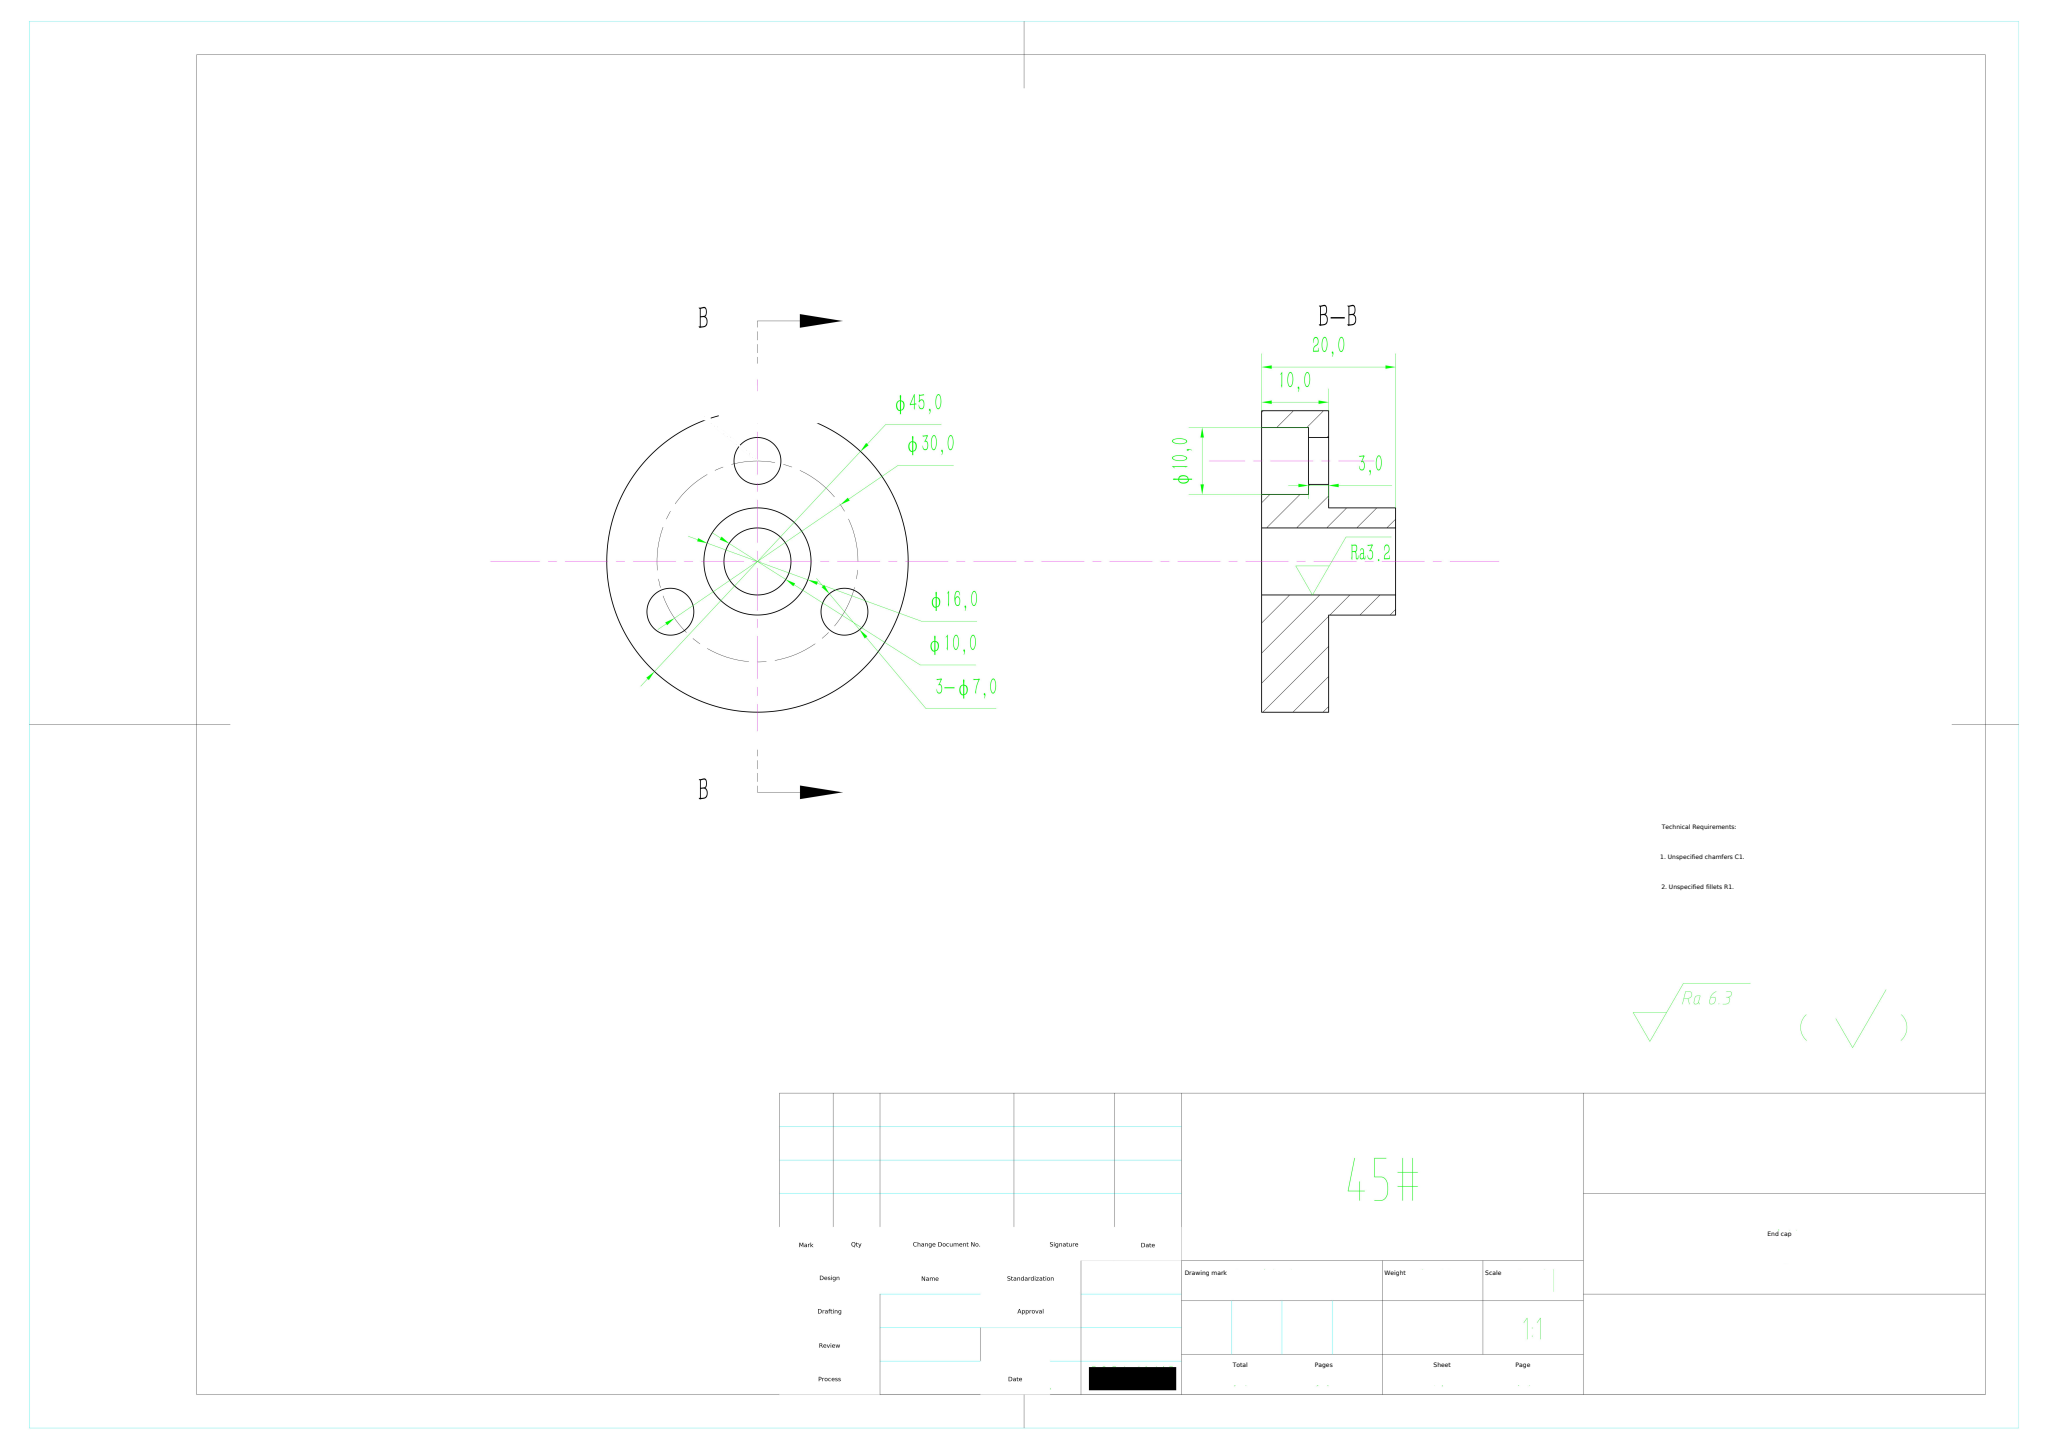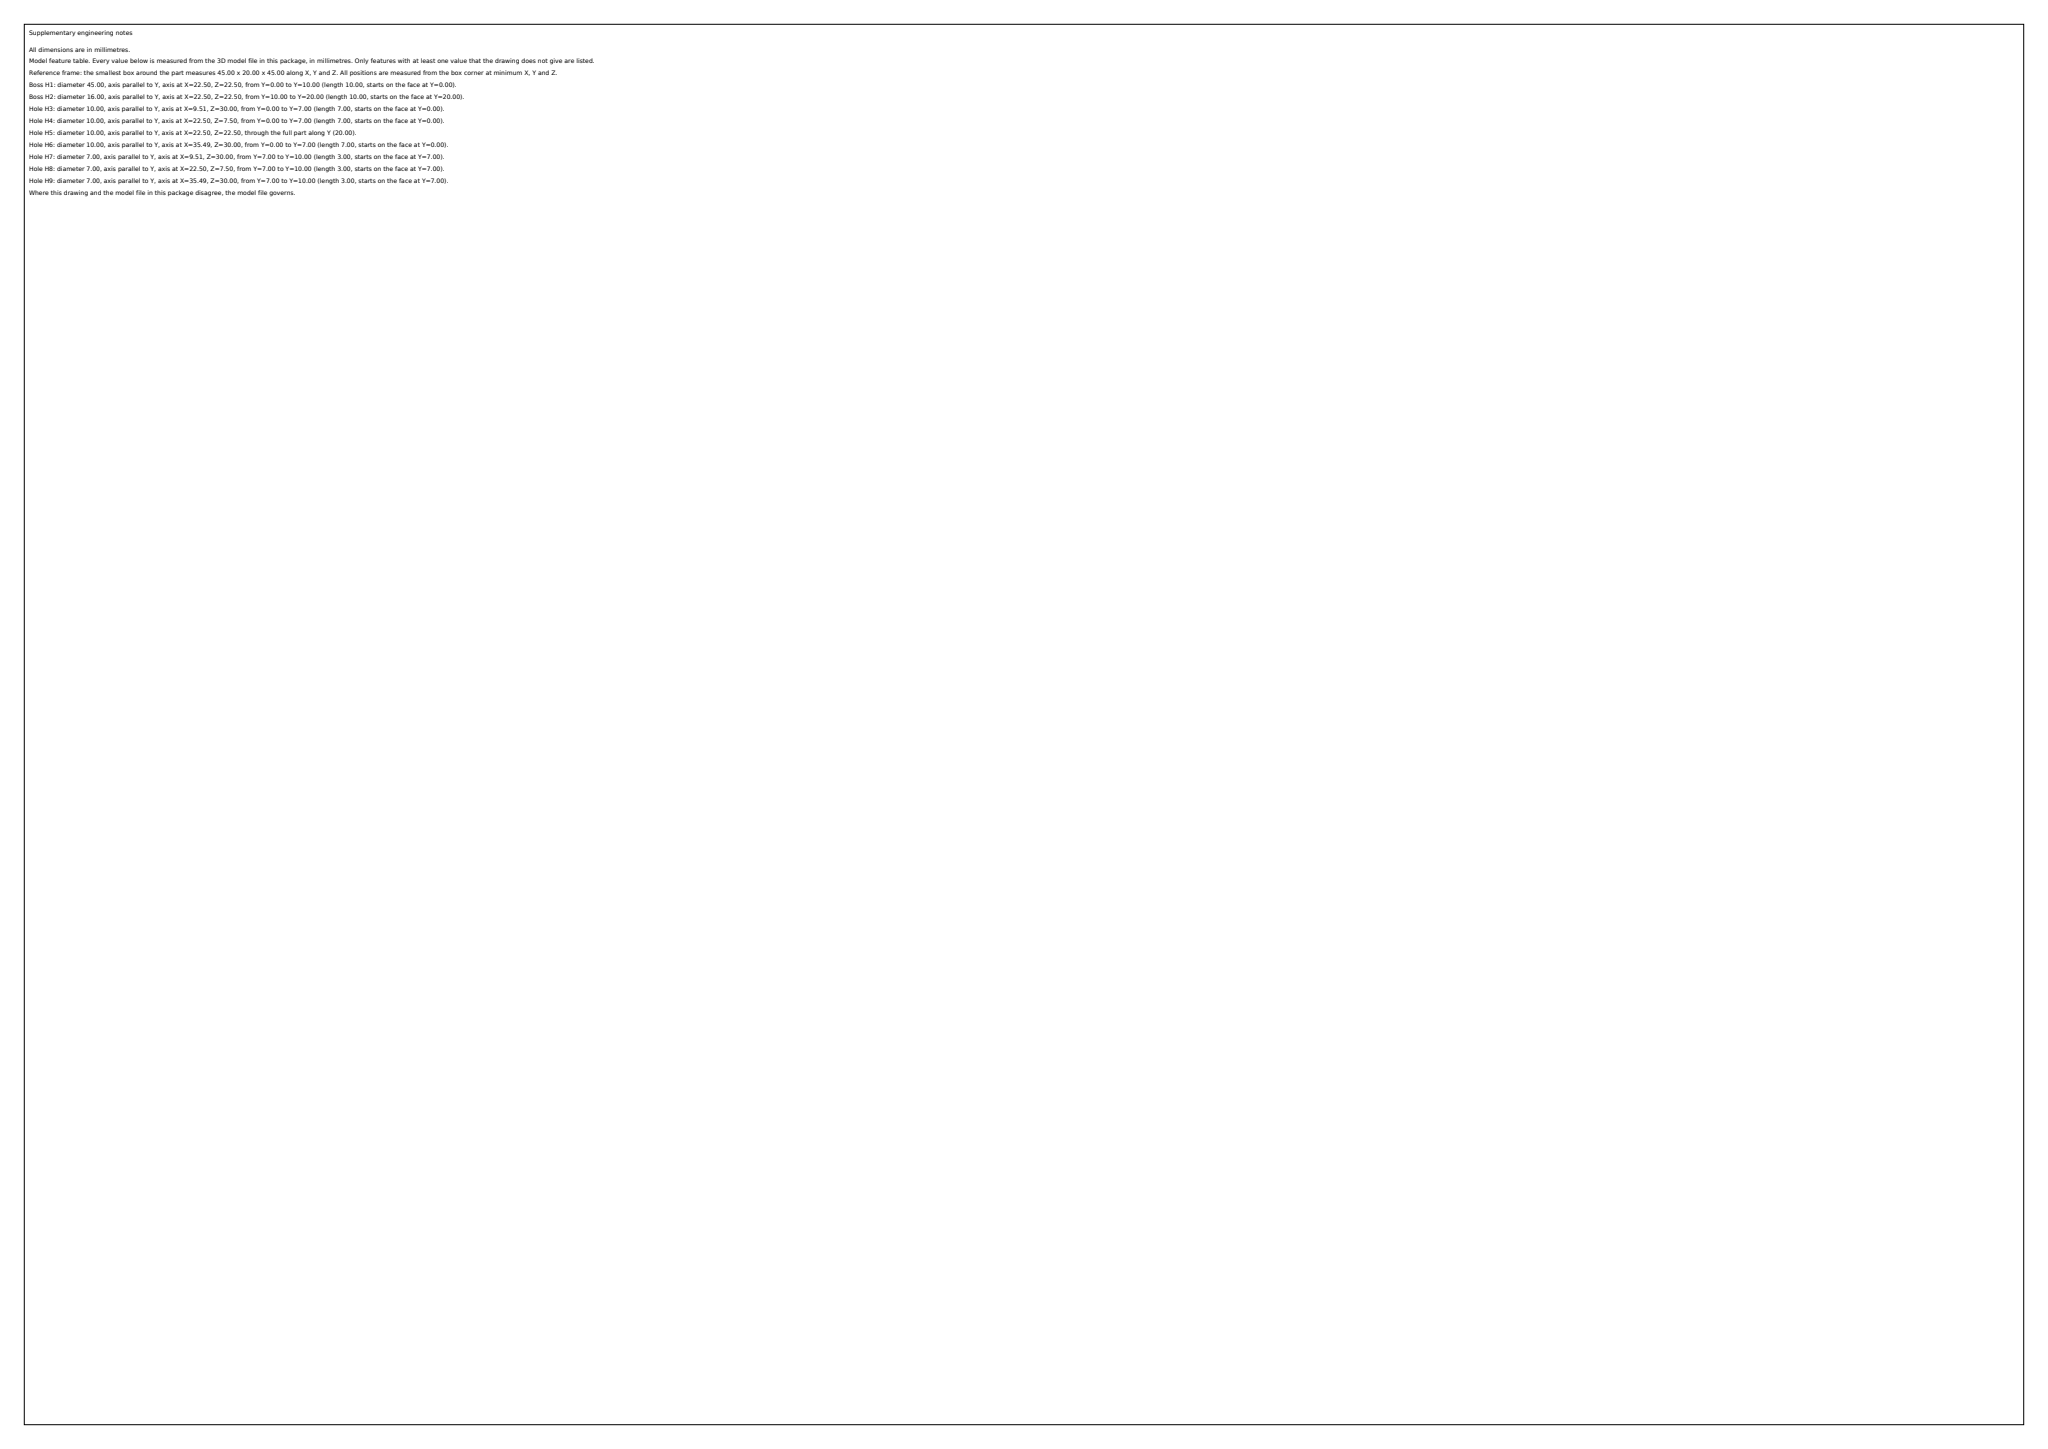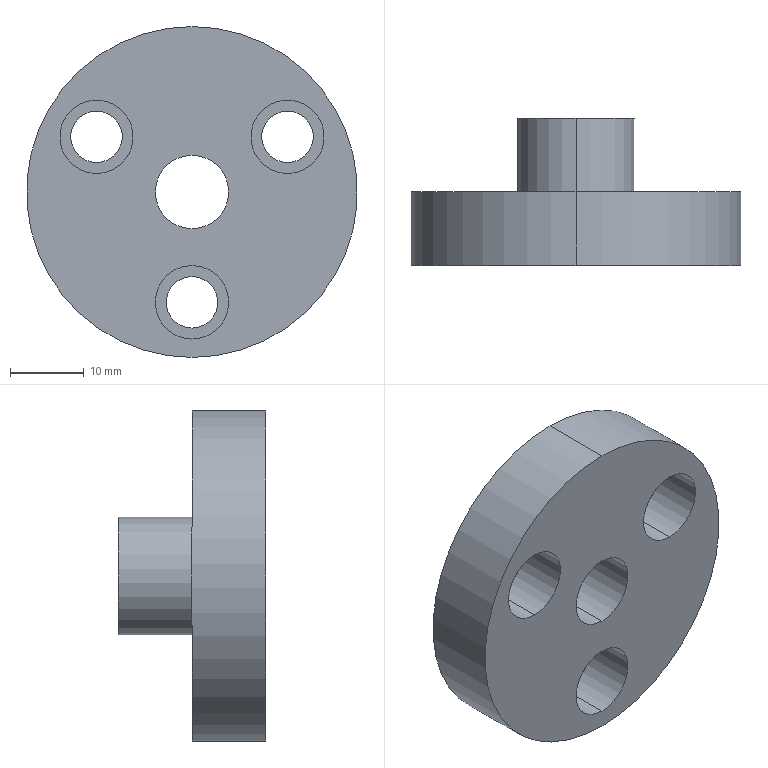Part | SolidWorks | mm | material 45# | 1 solid | 24 faces | box 45 x 20 x 45 mm | volume 14348 mm3 | cylinder 18 | plane 6 | commonest cylinder face diameters 10 x8 7 x6 16 x2 45 x2
build123d program:
from build123d import *

# Parameters (mm, degrees)
SKETCH1_R           = 22.5
BOSS_EXTRUDE1_DEPTH = 10
SKETCH2_R           = 8
BOSS_EXTRUDE2_DEPTH = 10
SKETCH3_R           = 3.5
CUT_EXTRUDE1_DEPTH  = 34.354
SKETCH4_R           = 5
CUT_EXTRUDE2_DEPTH  = 38.583
SKETCH5_R           = 5
CUT_EXTRUDE3_DEPTH  = 7


with BuildPart() as part:
    # Sketch1 → Boss-Extrude1 (new body)
    with BuildSketch(Plane(origin=(0, 0, 0), x_dir=(1, 0, 0), z_dir=(0, 1, 0))):
        with Locations(Location((0, 0, 0), (0, 0, 270))):
            Circle(SKETCH1_R)
    extrude(amount=BOSS_EXTRUDE1_DEPTH)

    # Sketch2 → Boss-Extrude2 (add)
    with BuildSketch(Plane(origin=(0, 10, 0), x_dir=(1, 0, 0), z_dir=(0, 1, 0))):
        with Locations(Location((0, 0, 0), (0, 0, 270))):
            Circle(SKETCH2_R)
    extrude(amount=BOSS_EXTRUDE2_DEPTH)

    # Sketch3 → Cut-Extrude1 (cut, through all)
    with BuildSketch(Plane(origin=(0, 10, 0), x_dir=(1, 0, 0), z_dir=(0, 1, 0))):
        with Locations(Location((0, 15, 0), (0, 0, 270))):
            Circle(SKETCH3_R)
        with Locations(Location((12.99, -7.5, 0), (0, 0, 270))):
            Circle(SKETCH3_R)
        with Locations(Location((-12.99, -7.5, 0), (0, 0, 270))):
            Circle(SKETCH3_R)
    extrude(amount=-CUT_EXTRUDE1_DEPTH, mode=Mode.SUBTRACT)

    # Sketch4 → Cut-Extrude2 (cut, through all)
    with BuildSketch(Plane(origin=(0, 20, 0), x_dir=(1, 0, 0), z_dir=(0, 1, 0))):
        with Locations(Location((0, 0, 0), (0, 0, 270))):
            Circle(SKETCH4_R)
    extrude(amount=-CUT_EXTRUDE2_DEPTH, mode=Mode.SUBTRACT)

    # Sketch5 → Cut-Extrude3 (cut)
    with BuildSketch(Plane.XZ):
        with Locations(Location((12.99, 7.5, 0), (0, 0, 270))):
            Circle(SKETCH5_R)
        with Locations(Location((0, -15, 0), (0, 0, 270))):
            Circle(SKETCH5_R)
        with Locations(Location((-12.99, 7.5, 0), (0, 0, 270))):
            Circle(SKETCH5_R)
    extrude(amount=-CUT_EXTRUDE3_DEPTH, mode=Mode.SUBTRACT)


solid = part.part
STEP:
#1=CARTESIAN_POINT('',(-12.99,7.,12.5));
#2=VERTEX_POINT('',#1);
#3=CARTESIAN_POINT('',(-12.99,7.,2.5));
#4=VERTEX_POINT('',#3);
#5=CARTESIAN_POINT('',(-12.99,7.,7.5));
#6=DIRECTION('',(0.,-1.,0.));
#7=DIRECTION('',(0.,0.,-1.));
#8=AXIS2_PLACEMENT_3D('',#5,#6,#7);
#9=CIRCLE('',#8,5.);
#10=EDGE_CURVE('',#2,#4,#9,.T.);
#11=ORIENTED_EDGE('',*,*,#10,.F.);
#12=CARTESIAN_POINT('',(-12.99,0.,12.5));
#13=VERTEX_POINT('',#12);
#14=CARTESIAN_POINT('',(-12.99,7.,12.5));
#15=DIRECTION('',(0.,-1.,0.));
#16=VECTOR('',#15,1000.);
#17=LINE('',#14,#16);
#18=EDGE_CURVE('',#2,#13,#17,.T.);
#19=ORIENTED_EDGE('',*,*,#18,.T.);
#20=CARTESIAN_POINT('',(-12.99,0.,2.5));
#21=VERTEX_POINT('',#20);
#22=CARTESIAN_POINT('',(-12.99,0.,7.5));
#23=DIRECTION('',(0.,-1.,0.));
#24=DIRECTION('',(0.,0.,-1.));
#25=AXIS2_PLACEMENT_3D('',#22,#23,#24);
#26=CIRCLE('',#25,5.);
#27=EDGE_CURVE('',#13,#21,#26,.T.);
#28=ORIENTED_EDGE('',*,*,#27,.T.);
#29=CARTESIAN_POINT('',(-12.99,7.,2.5));
#30=DIRECTION('',(0.,-1.,0.));
#31=VECTOR('',#30,1000.);
#32=LINE('',#29,#31);
#33=EDGE_CURVE('',#4,#21,#32,.T.);
#34=ORIENTED_EDGE('',*,*,#33,.F.);
#35=EDGE_LOOP('',(#11,#19,#28,#34));
#36=FACE_OUTER_BOUND('',#35,.T.);
#37=CARTESIAN_POINT('',(-12.99,7.,7.5));
#38=DIRECTION('',(0.,-1.,0.));
#39=DIRECTION('',(0.,0.,-1.));
#40=AXIS2_PLACEMENT_3D('',#37,#38,#39);
#41=CYLINDRICAL_SURFACE('',#40,5.);
#42=ADVANCED_FACE('',(#36),#41,.F.);
#43=CARTESIAN_POINT('',(12.99,7.,12.5));
#44=VERTEX_POINT('',#43);
#45=CARTESIAN_POINT('',(12.99,7.,2.5));
#46=VERTEX_POINT('',#45);
#47=CARTESIAN_POINT('',(12.99,7.,7.5));
#48=DIRECTION('',(0.,-1.,0.));
#49=DIRECTION('',(0.,0.,-1.));
#50=AXIS2_PLACEMENT_3D('',#47,#48,#49);
#51=CIRCLE('',#50,5.);
#52=EDGE_CURVE('',#44,#46,#51,.T.);
#53=ORIENTED_EDGE('',*,*,#52,.F.);
#54=CARTESIAN_POINT('',(12.99,0.,12.5));
#55=VERTEX_POINT('',#54);
#56=CARTESIAN_POINT('',(12.99,7.,12.5));
#57=DIRECTION('',(0.,-1.,0.));
#58=VECTOR('',#57,1000.);
#59=LINE('',#56,#58);
#60=EDGE_CURVE('',#44,#55,#59,.T.);
#61=ORIENTED_EDGE('',*,*,#60,.T.);
#62=CARTESIAN_POINT('',(12.99,0.,2.5));
#63=VERTEX_POINT('',#62);
#64=CARTESIAN_POINT('',(12.99,0.,7.5));
#65=DIRECTION('',(0.,-1.,0.));
#66=DIRECTION('',(0.,0.,-1.));
#67=AXIS2_PLACEMENT_3D('',#64,#65,#66);
#68=CIRCLE('',#67,5.);
#69=EDGE_CURVE('',#55,#63,#68,.T.);
#70=ORIENTED_EDGE('',*,*,#69,.T.);
#71=CARTESIAN_POINT('',(12.99,7.,2.5));
#72=DIRECTION('',(0.,-1.,0.));
#73=VECTOR('',#72,1000.);
#74=LINE('',#71,#73);
#75=EDGE_CURVE('',#46,#63,#74,.T.);
#76=ORIENTED_EDGE('',*,*,#75,.F.);
#77=EDGE_LOOP('',(#53,#61,#70,#76));
#78=FACE_OUTER_BOUND('',#77,.T.);
#79=CARTESIAN_POINT('',(12.99,7.,7.5));
#80=DIRECTION('',(0.,-1.,0.));
#81=DIRECTION('',(0.,0.,-1.));
#82=AXIS2_PLACEMENT_3D('',#79,#80,#81);
#83=CYLINDRICAL_SURFACE('',#82,5.);
#84=ADVANCED_FACE('',(#78),#83,.F.);
#85=CARTESIAN_POINT('',(-0.,7.,-10.));
#86=VERTEX_POINT('',#85);
#87=CARTESIAN_POINT('',(-0.,7.,-20.));
#88=VERTEX_POINT('',#87);
#89=CARTESIAN_POINT('',(-0.,7.,-15.));
#90=DIRECTION('',(0.,-1.,0.));
#91=DIRECTION('',(0.,0.,-1.));
#92=AXIS2_PLACEMENT_3D('',#89,#90,#91);
#93=CIRCLE('',#92,5.);
#94=EDGE_CURVE('',#86,#88,#93,.T.);
#95=ORIENTED_EDGE('',*,*,#94,.F.);
#96=CARTESIAN_POINT('',(-0.,0.,-10.));
#97=VERTEX_POINT('',#96);
#98=CARTESIAN_POINT('',(-0.,7.,-10.));
#99=DIRECTION('',(0.,-1.,0.));
#100=VECTOR('',#99,1000.);
#101=LINE('',#98,#100);
#102=EDGE_CURVE('',#86,#97,#101,.T.);
#103=ORIENTED_EDGE('',*,*,#102,.T.);
#104=CARTESIAN_POINT('',(-0.,0.,-20.));
#105=VERTEX_POINT('',#104);
#106=CARTESIAN_POINT('',(-0.,0.,-15.));
#107=DIRECTION('',(0.,-1.,0.));
#108=DIRECTION('',(0.,0.,-1.));
#109=AXIS2_PLACEMENT_3D('',#106,#107,#108);
#110=CIRCLE('',#109,5.);
#111=EDGE_CURVE('',#97,#105,#110,.T.);
#112=ORIENTED_EDGE('',*,*,#111,.T.);
#113=CARTESIAN_POINT('',(-0.,7.,-20.));
#114=DIRECTION('',(0.,-1.,0.));
#115=VECTOR('',#114,1000.);
#116=LINE('',#113,#115);
#117=EDGE_CURVE('',#88,#105,#116,.T.);
#118=ORIENTED_EDGE('',*,*,#117,.F.);
#119=EDGE_LOOP('',(#95,#103,#112,#118));
#120=FACE_OUTER_BOUND('',#119,.T.);
#121=CARTESIAN_POINT('',(-0.,7.,-15.));
#122=DIRECTION('',(0.,-1.,0.));
#123=DIRECTION('',(0.,0.,-1.));
#124=AXIS2_PLACEMENT_3D('',#121,#122,#123);
#125=CYLINDRICAL_SURFACE('',#124,5.);
#126=ADVANCED_FACE('',(#120),#125,.F.);
#127=CARTESIAN_POINT('',(0.,0.,-5.));
#128=VERTEX_POINT('',#127);
#129=CARTESIAN_POINT('',(0.,0.,5.));
#130=VERTEX_POINT('',#129);
#131=CARTESIAN_POINT('',(0.,0.,0.));
#132=DIRECTION('',(0.,1.,0.));
#133=DIRECTION('',(0.,0.,1.));
#134=AXIS2_PLACEMENT_3D('',#131,#132,#133);
#135=CIRCLE('',#134,5.);
#136=EDGE_CURVE('',#128,#130,#135,.T.);
#137=ORIENTED_EDGE('',*,*,#136,.F.);
#138=CARTESIAN_POINT('',(0.,20.,-5.));
#139=VERTEX_POINT('',#138);
#140=CARTESIAN_POINT('',(0.,0.,-5.));
#141=DIRECTION('',(0.,1.,0.));
#142=VECTOR('',#141,1000.);
#143=LINE('',#140,#142);
#144=EDGE_CURVE('',#128,#139,#143,.T.);
#145=ORIENTED_EDGE('',*,*,#144,.T.);
#146=CARTESIAN_POINT('',(0.,20.,5.));
#147=VERTEX_POINT('',#146);
#148=CARTESIAN_POINT('',(0.,20.,0.));
#149=DIRECTION('',(0.,1.,0.));
#150=DIRECTION('',(0.,0.,1.));
#151=AXIS2_PLACEMENT_3D('',#148,#149,#150);
#152=CIRCLE('',#151,5.);
#153=EDGE_CURVE('',#139,#147,#152,.T.);
#154=ORIENTED_EDGE('',*,*,#153,.T.);
#155=CARTESIAN_POINT('',(0.,0.,5.));
#156=DIRECTION('',(0.,1.,0.));
#157=VECTOR('',#156,1000.);
#158=LINE('',#155,#157);
#159=EDGE_CURVE('',#130,#147,#158,.T.);
#160=ORIENTED_EDGE('',*,*,#159,.F.);
#161=EDGE_LOOP('',(#137,#145,#154,#160));
#162=FACE_OUTER_BOUND('',#161,.T.);
#163=CARTESIAN_POINT('',(0.,0.,0.));
#164=DIRECTION('',(0.,1.,0.));
#165=DIRECTION('',(0.,0.,1.));
#166=AXIS2_PLACEMENT_3D('',#163,#164,#165);
#167=CYLINDRICAL_SURFACE('',#166,5.);
#168=ADVANCED_FACE('',(#162),#167,.F.);
#169=CARTESIAN_POINT('',(0.,20.,8.));
#170=VERTEX_POINT('',#169);
#171=CARTESIAN_POINT('',(0.,20.,-8.));
#172=VERTEX_POINT('',#171);
#173=CARTESIAN_POINT('',(0.,20.,0.));
#174=DIRECTION('',(0.,1.,0.));
#175=DIRECTION('',(0.,0.,1.));
#176=AXIS2_PLACEMENT_3D('',#173,#174,#175);
#177=CIRCLE('',#176,8.);
#178=EDGE_CURVE('',#170,#172,#177,.T.);
#179=ORIENTED_EDGE('',*,*,#178,.F.);
#180=CARTESIAN_POINT('',(0.,10.,8.));
#181=VERTEX_POINT('',#180);
#182=CARTESIAN_POINT('',(0.,20.,8.));
#183=DIRECTION('',(0.,-1.,0.));
#184=VECTOR('',#183,1000.);
#185=LINE('',#182,#184);
#186=EDGE_CURVE('',#170,#181,#185,.T.);
#187=ORIENTED_EDGE('',*,*,#186,.T.);
#188=CARTESIAN_POINT('',(0.,10.,-8.));
#189=VERTEX_POINT('',#188);
#190=CARTESIAN_POINT('',(0.,10.,0.));
#191=DIRECTION('',(0.,1.,0.));
#192=DIRECTION('',(0.,0.,1.));
#193=AXIS2_PLACEMENT_3D('',#190,#191,#192);
#194=CIRCLE('',#193,8.);
#195=EDGE_CURVE('',#181,#189,#194,.T.);
#196=ORIENTED_EDGE('',*,*,#195,.T.);
#197=CARTESIAN_POINT('',(0.,20.,-8.));
#198=DIRECTION('',(0.,-1.,0.));
#199=VECTOR('',#198,1000.);
#200=LINE('',#197,#199);
#201=EDGE_CURVE('',#172,#189,#200,.T.);
#202=ORIENTED_EDGE('',*,*,#201,.F.);
#203=EDGE_LOOP('',(#179,#187,#196,#202));
#204=FACE_OUTER_BOUND('',#203,.T.);
#205=CARTESIAN_POINT('',(0.,20.,0.));
#206=DIRECTION('',(0.,-1.,0.));
#207=DIRECTION('',(0.,0.,-1.));
#208=AXIS2_PLACEMENT_3D('',#205,#206,#207);
#209=CYLINDRICAL_SURFACE('',#208,8.);
#210=ADVANCED_FACE('',(#204),#209,.T.);
#211=CARTESIAN_POINT('',(0.,10.,22.5));
#212=VERTEX_POINT('',#211);
#213=CARTESIAN_POINT('',(0.,10.,-22.5));
#214=VERTEX_POINT('',#213);
#215=CARTESIAN_POINT('',(0.,10.,0.));
#216=DIRECTION('',(0.,1.,0.));
#217=DIRECTION('',(0.,0.,1.));
#218=AXIS2_PLACEMENT_3D('',#215,#216,#217);
#219=CIRCLE('',#218,22.5);
#220=EDGE_CURVE('',#212,#214,#219,.T.);
#221=ORIENTED_EDGE('',*,*,#220,.F.);
#222=CARTESIAN_POINT('',(0.,0.,22.5));
#223=VERTEX_POINT('',#222);
#224=CARTESIAN_POINT('',(0.,10.,22.5));
#225=DIRECTION('',(0.,-1.,0.));
#226=VECTOR('',#225,1000.);
#227=LINE('',#224,#226);
#228=EDGE_CURVE('',#212,#223,#227,.T.);
#229=ORIENTED_EDGE('',*,*,#228,.T.);
#230=CARTESIAN_POINT('',(0.,0.,-22.5));
#231=VERTEX_POINT('',#230);
#232=CARTESIAN_POINT('',(0.,0.,0.));
#233=DIRECTION('',(0.,1.,0.));
#234=DIRECTION('',(0.,0.,1.));
#235=AXIS2_PLACEMENT_3D('',#232,#233,#234);
#236=CIRCLE('',#235,22.5);
#237=EDGE_CURVE('',#223,#231,#236,.T.);
#238=ORIENTED_EDGE('',*,*,#237,.T.);
#239=CARTESIAN_POINT('',(0.,10.,-22.5));
#240=DIRECTION('',(0.,-1.,0.));
#241=VECTOR('',#240,1000.);
#242=LINE('',#239,#241);
#243=EDGE_CURVE('',#214,#231,#242,.T.);
#244=ORIENTED_EDGE('',*,*,#243,.F.);
#245=EDGE_LOOP('',(#221,#229,#238,#244));
#246=FACE_OUTER_BOUND('',#245,.T.);
#247=CARTESIAN_POINT('',(0.,10.,0.));
#248=DIRECTION('',(0.,-1.,0.));
#249=DIRECTION('',(0.,0.,-1.));
#250=AXIS2_PLACEMENT_3D('',#247,#248,#249);
#251=CYLINDRICAL_SURFACE('',#250,22.5);
#252=ADVANCED_FACE('',(#246),#251,.T.);
#253=CARTESIAN_POINT('',(0.,7.,-18.5));
#254=VERTEX_POINT('',#253);
#255=CARTESIAN_POINT('',(0.,7.,-11.5));
#256=VERTEX_POINT('',#255);
#257=CARTESIAN_POINT('',(0.,7.,-15.));
#258=DIRECTION('',(0.,1.,0.));
#259=DIRECTION('',(0.,0.,-1.));
#260=AXIS2_PLACEMENT_3D('',#257,#258,#259);
#261=CIRCLE('',#260,3.5);
#262=EDGE_CURVE('',#254,#256,#261,.T.);
#263=ORIENTED_EDGE('',*,*,#262,.F.);
#264=CARTESIAN_POINT('',(0.,10.,-18.5));
#265=VERTEX_POINT('',#264);
#266=CARTESIAN_POINT('',(0.,0.,-18.5));
#267=DIRECTION('',(0.,1.,0.));
#268=VECTOR('',#267,1000.);
#269=LINE('',#266,#268);
#270=EDGE_CURVE('',#254,#265,#269,.T.);
#271=ORIENTED_EDGE('',*,*,#270,.T.);
#272=CARTESIAN_POINT('',(0.,10.,-11.5));
#273=VERTEX_POINT('',#272);
#274=CARTESIAN_POINT('',(0.,10.,-15.));
#275=DIRECTION('',(0.,1.,0.));
#276=DIRECTION('',(0.,0.,1.));
#277=AXIS2_PLACEMENT_3D('',#274,#275,#276);
#278=CIRCLE('',#277,3.5);
#279=EDGE_CURVE('',#265,#273,#278,.T.);
#280=ORIENTED_EDGE('',*,*,#279,.T.);
#281=CARTESIAN_POINT('',(0.,0.,-11.5));
#282=DIRECTION('',(0.,1.,0.));
#283=VECTOR('',#282,1000.);
#284=LINE('',#281,#283);
#285=EDGE_CURVE('',#256,#273,#284,.T.);
#286=ORIENTED_EDGE('',*,*,#285,.F.);
#287=EDGE_LOOP('',(#263,#271,#280,#286));
#288=FACE_OUTER_BOUND('',#287,.T.);
#289=CARTESIAN_POINT('',(0.,0.,-15.));
#290=DIRECTION('',(0.,1.,0.));
#291=DIRECTION('',(0.,0.,1.));
#292=AXIS2_PLACEMENT_3D('',#289,#290,#291);
#293=CYLINDRICAL_SURFACE('',#292,3.5);
#294=ADVANCED_FACE('',(#288),#293,.F.);
#295=CARTESIAN_POINT('',(12.99,7.,4.));
#296=VERTEX_POINT('',#295);
#297=CARTESIAN_POINT('',(12.99,7.,11.));
#298=VERTEX_POINT('',#297);
#299=CARTESIAN_POINT('',(12.99,7.,7.5));
#300=DIRECTION('',(0.,1.,0.));
#301=DIRECTION('',(0.,0.,-1.));
#302=AXIS2_PLACEMENT_3D('',#299,#300,#301);
#303=CIRCLE('',#302,3.5);
#304=EDGE_CURVE('',#296,#298,#303,.T.);
#305=ORIENTED_EDGE('',*,*,#304,.F.);
#306=CARTESIAN_POINT('',(12.99,10.,4.));
#307=VERTEX_POINT('',#306);
#308=CARTESIAN_POINT('',(12.99,0.,4.));
#309=DIRECTION('',(0.,1.,0.));
#310=VECTOR('',#309,1000.);
#311=LINE('',#308,#310);
#312=EDGE_CURVE('',#296,#307,#311,.T.);
#313=ORIENTED_EDGE('',*,*,#312,.T.);
#314=CARTESIAN_POINT('',(12.99,10.,11.));
#315=VERTEX_POINT('',#314);
#316=CARTESIAN_POINT('',(12.99,10.,7.5));
#317=DIRECTION('',(0.,1.,0.));
#318=DIRECTION('',(0.,0.,1.));
#319=AXIS2_PLACEMENT_3D('',#316,#317,#318);
#320=CIRCLE('',#319,3.5);
#321=EDGE_CURVE('',#307,#315,#320,.T.);
#322=ORIENTED_EDGE('',*,*,#321,.T.);
#323=CARTESIAN_POINT('',(12.99,0.,11.));
#324=DIRECTION('',(0.,1.,0.));
#325=VECTOR('',#324,1000.);
#326=LINE('',#323,#325);
#327=EDGE_CURVE('',#298,#315,#326,.T.);
#328=ORIENTED_EDGE('',*,*,#327,.F.);
#329=EDGE_LOOP('',(#305,#313,#322,#328));
#330=FACE_OUTER_BOUND('',#329,.T.);
#331=CARTESIAN_POINT('',(12.99,0.,7.5));
#332=DIRECTION('',(0.,1.,0.));
#333=DIRECTION('',(0.,0.,1.));
#334=AXIS2_PLACEMENT_3D('',#331,#332,#333);
#335=CYLINDRICAL_SURFACE('',#334,3.5);
#336=ADVANCED_FACE('',(#330),#335,.F.);
#337=CARTESIAN_POINT('',(-12.99,7.,4.));
#338=VERTEX_POINT('',#337);
#339=CARTESIAN_POINT('',(-12.99,7.,11.));
#340=VERTEX_POINT('',#339);
#341=CARTESIAN_POINT('',(-12.99,7.,7.5));
#342=DIRECTION('',(0.,1.,0.));
#343=DIRECTION('',(0.,0.,-1.));
#344=AXIS2_PLACEMENT_3D('',#341,#342,#343);
#345=CIRCLE('',#344,3.5);
#346=EDGE_CURVE('',#338,#340,#345,.T.);
#347=ORIENTED_EDGE('',*,*,#346,.F.);
#348=CARTESIAN_POINT('',(-12.99,10.,4.));
#349=VERTEX_POINT('',#348);
#350=CARTESIAN_POINT('',(-12.99,0.,4.));
#351=DIRECTION('',(0.,1.,0.));
#352=VECTOR('',#351,1000.);
#353=LINE('',#350,#352);
#354=EDGE_CURVE('',#338,#349,#353,.T.);
#355=ORIENTED_EDGE('',*,*,#354,.T.);
#356=CARTESIAN_POINT('',(-12.99,10.,11.));
#357=VERTEX_POINT('',#356);
#358=CARTESIAN_POINT('',(-12.99,10.,7.5));
#359=DIRECTION('',(0.,1.,0.));
#360=DIRECTION('',(0.,0.,1.));
#361=AXIS2_PLACEMENT_3D('',#358,#359,#360);
#362=CIRCLE('',#361,3.5);
#363=EDGE_CURVE('',#349,#357,#362,.T.);
#364=ORIENTED_EDGE('',*,*,#363,.T.);
#365=CARTESIAN_POINT('',(-12.99,0.,11.));
#366=DIRECTION('',(0.,1.,0.));
#367=VECTOR('',#366,1000.);
#368=LINE('',#365,#367);
#369=EDGE_CURVE('',#340,#357,#368,.T.);
#370=ORIENTED_EDGE('',*,*,#369,.F.);
#371=EDGE_LOOP('',(#347,#355,#364,#370));
#372=FACE_OUTER_BOUND('',#371,.T.);
#373=CARTESIAN_POINT('',(-12.99,0.,7.5));
#374=DIRECTION('',(0.,1.,0.));
#375=DIRECTION('',(0.,0.,1.));
#376=AXIS2_PLACEMENT_3D('',#373,#374,#375);
#377=CYLINDRICAL_SURFACE('',#376,3.5);
#378=ADVANCED_FACE('',(#372),#377,.F.);
#379=ORIENTED_EDGE('',*,*,#354,.F.);
#380=CARTESIAN_POINT('',(-12.99,7.,7.5));
#381=DIRECTION('',(0.,1.,0.));
#382=DIRECTION('',(0.,0.,-1.));
#383=AXIS2_PLACEMENT_3D('',#380,#381,#382);
#384=CIRCLE('',#383,3.5);
#385=EDGE_CURVE('',#340,#338,#384,.T.);
#386=ORIENTED_EDGE('',*,*,#385,.F.);
#387=ORIENTED_EDGE('',*,*,#369,.T.);
#388=CARTESIAN_POINT('',(-12.99,10.,7.5));
#389=DIRECTION('',(0.,1.,0.));
#390=DIRECTION('',(0.,0.,1.));
#391=AXIS2_PLACEMENT_3D('',#388,#389,#390);
#392=CIRCLE('',#391,3.5);
#393=EDGE_CURVE('',#357,#349,#392,.T.);
#394=ORIENTED_EDGE('',*,*,#393,.T.);
#395=EDGE_LOOP('',(#379,#386,#387,#394));
#396=FACE_OUTER_BOUND('',#395,.T.);
#397=CARTESIAN_POINT('',(-12.99,0.,7.5));
#398=DIRECTION('',(0.,1.,0.));
#399=DIRECTION('',(0.,0.,1.));
#400=AXIS2_PLACEMENT_3D('',#397,#398,#399);
#401=CYLINDRICAL_SURFACE('',#400,3.5);
#402=ADVANCED_FACE('',(#396),#401,.F.);
#403=ORIENTED_EDGE('',*,*,#312,.F.);
#404=CARTESIAN_POINT('',(12.99,7.,7.5));
#405=DIRECTION('',(0.,1.,0.));
#406=DIRECTION('',(0.,0.,-1.));
#407=AXIS2_PLACEMENT_3D('',#404,#405,#406);
#408=CIRCLE('',#407,3.5);
#409=EDGE_CURVE('',#298,#296,#408,.T.);
#410=ORIENTED_EDGE('',*,*,#409,.F.);
#411=ORIENTED_EDGE('',*,*,#327,.T.);
#412=CARTESIAN_POINT('',(12.99,10.,7.5));
#413=DIRECTION('',(0.,1.,0.));
#414=DIRECTION('',(0.,0.,1.));
#415=AXIS2_PLACEMENT_3D('',#412,#413,#414);
#416=CIRCLE('',#415,3.5);
#417=EDGE_CURVE('',#315,#307,#416,.T.);
#418=ORIENTED_EDGE('',*,*,#417,.T.);
#419=EDGE_LOOP('',(#403,#410,#411,#418));
#420=FACE_OUTER_BOUND('',#419,.T.);
#421=CARTESIAN_POINT('',(12.99,0.,7.5));
#422=DIRECTION('',(0.,1.,0.));
#423=DIRECTION('',(0.,0.,1.));
#424=AXIS2_PLACEMENT_3D('',#421,#422,#423);
#425=CYLINDRICAL_SURFACE('',#424,3.5);
#426=ADVANCED_FACE('',(#420),#425,.F.);
#427=ORIENTED_EDGE('',*,*,#270,.F.);
#428=CARTESIAN_POINT('',(0.,7.,-15.));
#429=DIRECTION('',(0.,1.,0.));
#430=DIRECTION('',(0.,0.,-1.));
#431=AXIS2_PLACEMENT_3D('',#428,#429,#430);
#432=CIRCLE('',#431,3.5);
#433=EDGE_CURVE('',#256,#254,#432,.T.);
#434=ORIENTED_EDGE('',*,*,#433,.F.);
#435=ORIENTED_EDGE('',*,*,#285,.T.);
#436=CARTESIAN_POINT('',(0.,10.,-15.));
#437=DIRECTION('',(0.,1.,0.));
#438=DIRECTION('',(0.,0.,1.));
#439=AXIS2_PLACEMENT_3D('',#436,#437,#438);
#440=CIRCLE('',#439,3.5);
#441=EDGE_CURVE('',#273,#265,#440,.T.);
#442=ORIENTED_EDGE('',*,*,#441,.T.);
#443=EDGE_LOOP('',(#427,#434,#435,#442));
#444=FACE_OUTER_BOUND('',#443,.T.);
#445=CARTESIAN_POINT('',(0.,0.,-15.));
#446=DIRECTION('',(0.,1.,0.));
#447=DIRECTION('',(0.,0.,1.));
#448=AXIS2_PLACEMENT_3D('',#445,#446,#447);
#449=CYLINDRICAL_SURFACE('',#448,3.5);
#450=ADVANCED_FACE('',(#444),#449,.F.);
#451=ORIENTED_EDGE('',*,*,#228,.F.);
#452=CARTESIAN_POINT('',(0.,10.,0.));
#453=DIRECTION('',(0.,1.,0.));
#454=DIRECTION('',(0.,0.,1.));
#455=AXIS2_PLACEMENT_3D('',#452,#453,#454);
#456=CIRCLE('',#455,22.5);
#457=EDGE_CURVE('',#214,#212,#456,.T.);
#458=ORIENTED_EDGE('',*,*,#457,.F.);
#459=ORIENTED_EDGE('',*,*,#243,.T.);
#460=CARTESIAN_POINT('',(0.,0.,0.));
#461=DIRECTION('',(0.,1.,0.));
#462=DIRECTION('',(0.,0.,1.));
#463=AXIS2_PLACEMENT_3D('',#460,#461,#462);
#464=CIRCLE('',#463,22.5);
#465=EDGE_CURVE('',#231,#223,#464,.T.);
#466=ORIENTED_EDGE('',*,*,#465,.T.);
#467=EDGE_LOOP('',(#451,#458,#459,#466));
#468=FACE_OUTER_BOUND('',#467,.T.);
#469=CARTESIAN_POINT('',(0.,10.,0.));
#470=DIRECTION('',(0.,-1.,0.));
#471=DIRECTION('',(0.,0.,-1.));
#472=AXIS2_PLACEMENT_3D('',#469,#470,#471);
#473=CYLINDRICAL_SURFACE('',#472,22.5);
#474=ADVANCED_FACE('',(#468),#473,.T.);
#475=ORIENTED_EDGE('',*,*,#441,.F.);
#476=ORIENTED_EDGE('',*,*,#279,.F.);
#477=EDGE_LOOP('',(#475,#476));
#478=FACE_BOUND('',#477,.T.);
#479=ORIENTED_EDGE('',*,*,#417,.F.);
#480=ORIENTED_EDGE('',*,*,#321,.F.);
#481=EDGE_LOOP('',(#479,#480));
#482=FACE_BOUND('',#481,.T.);
#483=ORIENTED_EDGE('',*,*,#393,.F.);
#484=ORIENTED_EDGE('',*,*,#363,.F.);
#485=EDGE_LOOP('',(#483,#484));
#486=FACE_BOUND('',#485,.T.);
#487=CARTESIAN_POINT('',(0.,10.,0.));
#488=DIRECTION('',(0.,1.,0.));
#489=DIRECTION('',(0.,0.,1.));
#490=AXIS2_PLACEMENT_3D('',#487,#488,#489);
#491=CIRCLE('',#490,8.);
#492=EDGE_CURVE('',#189,#181,#491,.T.);
#493=ORIENTED_EDGE('',*,*,#492,.F.);
#494=ORIENTED_EDGE('',*,*,#195,.F.);
#495=EDGE_LOOP('',(#493,#494));
#496=FACE_BOUND('',#495,.T.);
#497=ORIENTED_EDGE('',*,*,#457,.T.);
#498=ORIENTED_EDGE('',*,*,#220,.T.);
#499=EDGE_LOOP('',(#497,#498));
#500=FACE_OUTER_BOUND('',#499,.T.);
#501=CARTESIAN_POINT('',(0.,10.,0.));
#502=DIRECTION('',(0.,1.,0.));
#503=DIRECTION('',(0.,0.,1.));
#504=AXIS2_PLACEMENT_3D('',#501,#502,#503);
#505=PLANE('',#504);
#506=ADVANCED_FACE('',(#478,#482,#486,#496,#500),#505,.T.);
#507=CARTESIAN_POINT('',(12.99,0.,7.5));
#508=DIRECTION('',(0.,-1.,0.));
#509=DIRECTION('',(0.,0.,-1.));
#510=AXIS2_PLACEMENT_3D('',#507,#508,#509);
#511=CIRCLE('',#510,5.);
#512=EDGE_CURVE('',#63,#55,#511,.T.);
#513=ORIENTED_EDGE('',*,*,#512,.F.);
#514=ORIENTED_EDGE('',*,*,#69,.F.);
#515=EDGE_LOOP('',(#513,#514));
#516=FACE_BOUND('',#515,.T.);
#517=CARTESIAN_POINT('',(-0.,0.,-15.));
#518=DIRECTION('',(0.,-1.,0.));
#519=DIRECTION('',(0.,0.,-1.));
#520=AXIS2_PLACEMENT_3D('',#517,#518,#519);
#521=CIRCLE('',#520,5.);
#522=EDGE_CURVE('',#105,#97,#521,.T.);
#523=ORIENTED_EDGE('',*,*,#522,.F.);
#524=ORIENTED_EDGE('',*,*,#111,.F.);
#525=EDGE_LOOP('',(#523,#524));
#526=FACE_BOUND('',#525,.T.);
#527=CARTESIAN_POINT('',(-12.99,0.,7.5));
#528=DIRECTION('',(0.,-1.,0.));
#529=DIRECTION('',(0.,0.,-1.));
#530=AXIS2_PLACEMENT_3D('',#527,#528,#529);
#531=CIRCLE('',#530,5.);
#532=EDGE_CURVE('',#21,#13,#531,.T.);
#533=ORIENTED_EDGE('',*,*,#532,.F.);
#534=ORIENTED_EDGE('',*,*,#27,.F.);
#535=EDGE_LOOP('',(#533,#534));
#536=FACE_BOUND('',#535,.T.);
#537=CARTESIAN_POINT('',(0.,0.,0.));
#538=DIRECTION('',(0.,1.,0.));
#539=DIRECTION('',(0.,0.,1.));
#540=AXIS2_PLACEMENT_3D('',#537,#538,#539);
#541=CIRCLE('',#540,5.);
#542=EDGE_CURVE('',#130,#128,#541,.T.);
#543=ORIENTED_EDGE('',*,*,#542,.T.);
#544=ORIENTED_EDGE('',*,*,#136,.T.);
#545=EDGE_LOOP('',(#543,#544));
#546=FACE_BOUND('',#545,.T.);
#547=ORIENTED_EDGE('',*,*,#465,.F.);
#548=ORIENTED_EDGE('',*,*,#237,.F.);
#549=EDGE_LOOP('',(#547,#548));
#550=FACE_OUTER_BOUND('',#549,.T.);
#551=CARTESIAN_POINT('',(0.,0.,0.));
#552=DIRECTION('',(0.,1.,0.));
#553=DIRECTION('',(0.,0.,1.));
#554=AXIS2_PLACEMENT_3D('',#551,#552,#553);
#555=PLANE('',#554);
#556=ADVANCED_FACE('',(#516,#526,#536,#546,#550),#555,.F.);
#557=ORIENTED_EDGE('',*,*,#186,.F.);
#558=CARTESIAN_POINT('',(0.,20.,0.));
#559=DIRECTION('',(0.,1.,0.));
#560=DIRECTION('',(0.,0.,1.));
#561=AXIS2_PLACEMENT_3D('',#558,#559,#560);
#562=CIRCLE('',#561,8.);
#563=EDGE_CURVE('',#172,#170,#562,.T.);
#564=ORIENTED_EDGE('',*,*,#563,.F.);
#565=ORIENTED_EDGE('',*,*,#201,.T.);
#566=ORIENTED_EDGE('',*,*,#492,.T.);
#567=EDGE_LOOP('',(#557,#564,#565,#566));
#568=FACE_OUTER_BOUND('',#567,.T.);
#569=CARTESIAN_POINT('',(0.,20.,0.));
#570=DIRECTION('',(0.,-1.,0.));
#571=DIRECTION('',(0.,0.,-1.));
#572=AXIS2_PLACEMENT_3D('',#569,#570,#571);
#573=CYLINDRICAL_SURFACE('',#572,8.);
#574=ADVANCED_FACE('',(#568),#573,.T.);
#575=CARTESIAN_POINT('',(0.,20.,0.));
#576=DIRECTION('',(0.,1.,0.));
#577=DIRECTION('',(0.,0.,1.));
#578=AXIS2_PLACEMENT_3D('',#575,#576,#577);
#579=CIRCLE('',#578,5.);
#580=EDGE_CURVE('',#147,#139,#579,.T.);
#581=ORIENTED_EDGE('',*,*,#580,.F.);
#582=ORIENTED_EDGE('',*,*,#153,.F.);
#583=EDGE_LOOP('',(#581,#582));
#584=FACE_BOUND('',#583,.T.);
#585=ORIENTED_EDGE('',*,*,#563,.T.);
#586=ORIENTED_EDGE('',*,*,#178,.T.);
#587=EDGE_LOOP('',(#585,#586));
#588=FACE_OUTER_BOUND('',#587,.T.);
#589=CARTESIAN_POINT('',(0.,20.,0.));
#590=DIRECTION('',(0.,1.,0.));
#591=DIRECTION('',(0.,0.,1.));
#592=AXIS2_PLACEMENT_3D('',#589,#590,#591);
#593=PLANE('',#592);
#594=ADVANCED_FACE('',(#584,#588),#593,.T.);
#595=ORIENTED_EDGE('',*,*,#144,.F.);
#596=ORIENTED_EDGE('',*,*,#542,.F.);
#597=ORIENTED_EDGE('',*,*,#159,.T.);
#598=ORIENTED_EDGE('',*,*,#580,.T.);
#599=EDGE_LOOP('',(#595,#596,#597,#598));
#600=FACE_OUTER_BOUND('',#599,.T.);
#601=CARTESIAN_POINT('',(0.,0.,0.));
#602=DIRECTION('',(0.,1.,0.));
#603=DIRECTION('',(0.,0.,1.));
#604=AXIS2_PLACEMENT_3D('',#601,#602,#603);
#605=CYLINDRICAL_SURFACE('',#604,5.);
#606=ADVANCED_FACE('',(#600),#605,.F.);
#607=CARTESIAN_POINT('',(-0.,7.,-15.));
#608=DIRECTION('',(0.,-1.,0.));
#609=DIRECTION('',(0.,0.,-1.));
#610=AXIS2_PLACEMENT_3D('',#607,#608,#609);
#611=CIRCLE('',#610,5.);
#612=EDGE_CURVE('',#88,#86,#611,.T.);
#613=ORIENTED_EDGE('',*,*,#612,.T.);
#614=ORIENTED_EDGE('',*,*,#94,.T.);
#615=EDGE_LOOP('',(#613,#614));
#616=FACE_OUTER_BOUND('',#615,.T.);
#617=ORIENTED_EDGE('',*,*,#433,.T.);
#618=ORIENTED_EDGE('',*,*,#262,.T.);
#619=EDGE_LOOP('',(#617,#618));
#620=FACE_BOUND('',#619,.T.);
#621=CARTESIAN_POINT('',(-0.,7.,-15.));
#622=DIRECTION('',(0.,-1.,0.));
#623=DIRECTION('',(0.,0.,-1.));
#624=AXIS2_PLACEMENT_3D('',#621,#622,#623);
#625=PLANE('',#624);
#626=ADVANCED_FACE('',(#616,#620),#625,.T.);
#627=ORIENTED_EDGE('',*,*,#102,.F.);
#628=ORIENTED_EDGE('',*,*,#612,.F.);
#629=ORIENTED_EDGE('',*,*,#117,.T.);
#630=ORIENTED_EDGE('',*,*,#522,.T.);
#631=EDGE_LOOP('',(#627,#628,#629,#630));
#632=FACE_OUTER_BOUND('',#631,.T.);
#633=CARTESIAN_POINT('',(-0.,7.,-15.));
#634=DIRECTION('',(0.,-1.,0.));
#635=DIRECTION('',(0.,0.,-1.));
#636=AXIS2_PLACEMENT_3D('',#633,#634,#635);
#637=CYLINDRICAL_SURFACE('',#636,5.);
#638=ADVANCED_FACE('',(#632),#637,.F.);
#639=CARTESIAN_POINT('',(12.99,7.,7.5));
#640=DIRECTION('',(0.,-1.,0.));
#641=DIRECTION('',(0.,0.,-1.));
#642=AXIS2_PLACEMENT_3D('',#639,#640,#641);
#643=CIRCLE('',#642,5.);
#644=EDGE_CURVE('',#46,#44,#643,.T.);
#645=ORIENTED_EDGE('',*,*,#644,.T.);
#646=ORIENTED_EDGE('',*,*,#52,.T.);
#647=EDGE_LOOP('',(#645,#646));
#648=FACE_OUTER_BOUND('',#647,.T.);
#649=ORIENTED_EDGE('',*,*,#409,.T.);
#650=ORIENTED_EDGE('',*,*,#304,.T.);
#651=EDGE_LOOP('',(#649,#650));
#652=FACE_BOUND('',#651,.T.);
#653=CARTESIAN_POINT('',(12.99,7.,7.5));
#654=DIRECTION('',(0.,-1.,0.));
#655=DIRECTION('',(0.,0.,-1.));
#656=AXIS2_PLACEMENT_3D('',#653,#654,#655);
#657=PLANE('',#656);
#658=ADVANCED_FACE('',(#648,#652),#657,.T.);
#659=ORIENTED_EDGE('',*,*,#60,.F.);
#660=ORIENTED_EDGE('',*,*,#644,.F.);
#661=ORIENTED_EDGE('',*,*,#75,.T.);
#662=ORIENTED_EDGE('',*,*,#512,.T.);
#663=EDGE_LOOP('',(#659,#660,#661,#662));
#664=FACE_OUTER_BOUND('',#663,.T.);
#665=CARTESIAN_POINT('',(12.99,7.,7.5));
#666=DIRECTION('',(0.,-1.,0.));
#667=DIRECTION('',(0.,0.,-1.));
#668=AXIS2_PLACEMENT_3D('',#665,#666,#667);
#669=CYLINDRICAL_SURFACE('',#668,5.);
#670=ADVANCED_FACE('',(#664),#669,.F.);
#671=CARTESIAN_POINT('',(-12.99,7.,7.5));
#672=DIRECTION('',(0.,-1.,0.));
#673=DIRECTION('',(0.,0.,-1.));
#674=AXIS2_PLACEMENT_3D('',#671,#672,#673);
#675=CIRCLE('',#674,5.);
#676=EDGE_CURVE('',#4,#2,#675,.T.);
#677=ORIENTED_EDGE('',*,*,#676,.T.);
#678=ORIENTED_EDGE('',*,*,#10,.T.);
#679=EDGE_LOOP('',(#677,#678));
#680=FACE_OUTER_BOUND('',#679,.T.);
#681=ORIENTED_EDGE('',*,*,#385,.T.);
#682=ORIENTED_EDGE('',*,*,#346,.T.);
#683=EDGE_LOOP('',(#681,#682));
#684=FACE_BOUND('',#683,.T.);
#685=CARTESIAN_POINT('',(-12.99,7.,7.5));
#686=DIRECTION('',(0.,-1.,0.));
#687=DIRECTION('',(0.,0.,-1.));
#688=AXIS2_PLACEMENT_3D('',#685,#686,#687);
#689=PLANE('',#688);
#690=ADVANCED_FACE('',(#680,#684),#689,.T.);
#691=ORIENTED_EDGE('',*,*,#18,.F.);
#692=ORIENTED_EDGE('',*,*,#676,.F.);
#693=ORIENTED_EDGE('',*,*,#33,.T.);
#694=ORIENTED_EDGE('',*,*,#532,.T.);
#695=EDGE_LOOP('',(#691,#692,#693,#694));
#696=FACE_OUTER_BOUND('',#695,.T.);
#697=CARTESIAN_POINT('',(-12.99,7.,7.5));
#698=DIRECTION('',(0.,-1.,0.));
#699=DIRECTION('',(0.,0.,-1.));
#700=AXIS2_PLACEMENT_3D('',#697,#698,#699);
#701=CYLINDRICAL_SURFACE('',#700,5.);
#702=ADVANCED_FACE('',(#696),#701,.F.);
#703=CLOSED_SHELL('',(#42,#84,#126,#168,#210,#252,#294,#336,#378,#402,#426,#450,#474,#506,#556,#574,#594,#606,#626,#638,#658,#670,#690,#702));
#704=MANIFOLD_SOLID_BREP('',#703);
#705=CARTESIAN_POINT('',(0.,0.,0.));
#706=DIRECTION('',(0.,0.,1.));
#707=DIRECTION('',(1.,0.,0.));
#708=AXIS2_PLACEMENT_3D('',#705,#706,#707);
#709=(LENGTH_UNIT()NAMED_UNIT(*)SI_UNIT(.MILLI.,.METRE.));
#710=UNCERTAINTY_MEASURE_WITH_UNIT(LENGTH_MEASURE(0.00001),#709,'','');
#711=(NAMED_UNIT(*)PLANE_ANGLE_UNIT()SI_UNIT($,.RADIAN.));
#712=(NAMED_UNIT(*)SI_UNIT($,.STERADIAN.)SOLID_ANGLE_UNIT());
#713=(GEOMETRIC_REPRESENTATION_CONTEXT(3)GLOBAL_UNCERTAINTY_ASSIGNED_CONTEXT((#710))GLOBAL_UNIT_ASSIGNED_CONTEXT((#709,#711,#712))REPRESENTATION_CONTEXT('',''));
#714=ADVANCED_BREP_SHAPE_REPRESENTATION('',(#704,#708),#713);